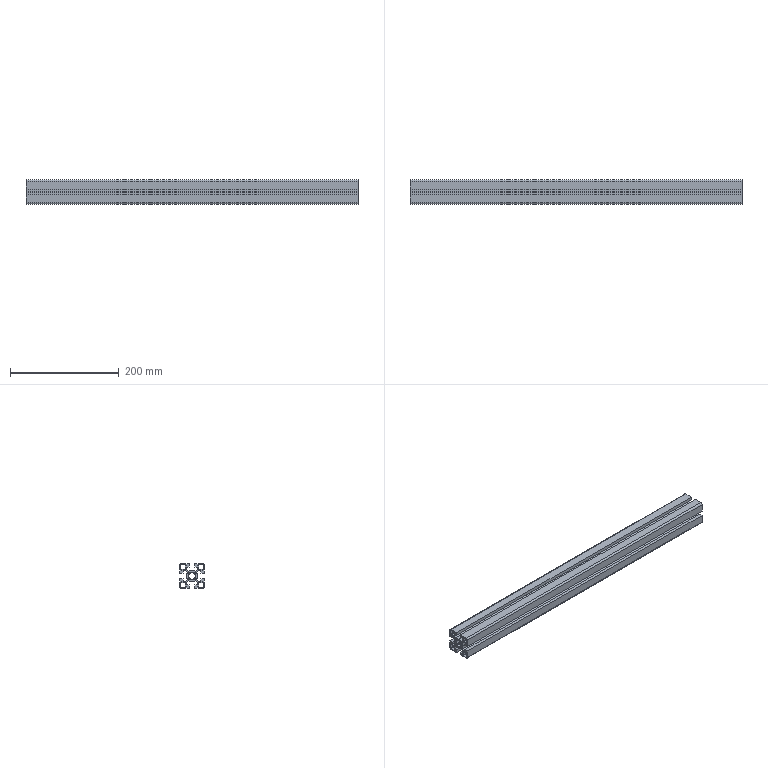Component | SolidWorks | 40-40AluminumProfileFrame-1_CAF8-4545-100FF-3-1 | 1 solid | 131 faces | volume 479445 mm3 | plane 82 | cylinder 49 | commonest cylinder face diameters 2 x18 3 x12 1 x10 12.5 x5 6 x4